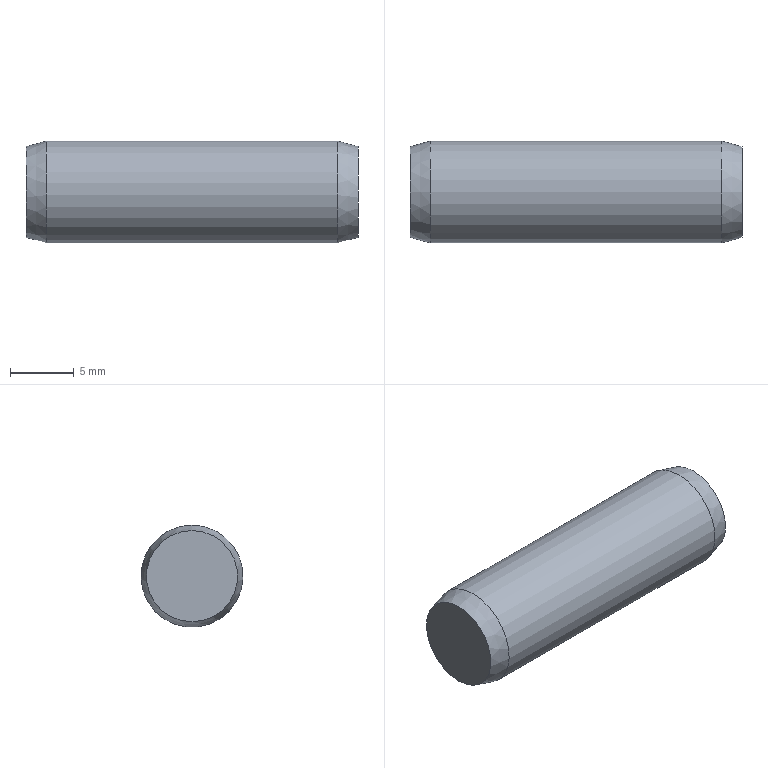Component | NX | GB-T119_1-2000_8X26 | 1 solid | 5 faces | box 26 x 8 x 8 mm | volume 1290 mm3 | plane 2 | cone 2 | cylinder 1 | commonest cylinder face diameters 8 x1
STEP:
#1=CARTESIAN_POINT('',(0.,0.,0.));
#2=DIRECTION('',(0.,0.,1.));
#3=DIRECTION('',(1.,0.,0.));
#4=AXIS2_PLACEMENT_3D('',#1,#2,#3);
#5=CARTESIAN_POINT('',(-11.39,31.008,-213.802));
#6=VERTEX_POINT('',#5);
#7=CARTESIAN_POINT('',(-11.39,31.008,-217.373));
#8=DIRECTION('',(-1.,0.,0.));
#9=DIRECTION('',(0.,0.,1.));
#10=AXIS2_PLACEMENT_3D('',#7,#8,#9);
#11=CIRCLE('',#10,3.571);
#12=CARTESIAN_POINT('',(-11.39,31.008,-217.373));
#13=DIRECTION('',(-1.,0.,0.));
#14=DIRECTION('',(0.,0.,1.));
#15=AXIS2_PLACEMENT_3D('',#12,#13,#14);
#16=PLANE('',#15);
#17=CARTESIAN_POINT('',(0.,0.));
#18=DIRECTION('',(1.,0.));
#19=AXIS2_PLACEMENT_2D('',#17,#18);
#20=CIRCLE('',#19,3.571);
#21=(GEOMETRIC_REPRESENTATION_CONTEXT(2)PARAMETRIC_REPRESENTATION_CONTEXT()REPRESENTATION_CONTEXT('',''));
#22=DEFINITIONAL_REPRESENTATION('',(#20),#21);
#23=PCURVE('',#16,#22);
#24=CARTESIAN_POINT('',(-11.39,31.008,-217.373));
#25=DIRECTION('',(1.,0.,0.));
#26=DIRECTION('',(0.,0.,-1.));
#27=AXIS2_PLACEMENT_3D('',#24,#25,#26);
#28=CONICAL_SURFACE('',#27,3.571,0.2618);
#29=CARTESIAN_POINT('',(9.425,-0.));
#30=DIRECTION('',(-1.,0.));
#31=VECTOR('',#30,1.);
#32=LINE('',#29,#31);
#33=(GEOMETRIC_REPRESENTATION_CONTEXT(2)PARAMETRIC_REPRESENTATION_CONTEXT()REPRESENTATION_CONTEXT('',''));
#34=DEFINITIONAL_REPRESENTATION('',(#32),#33);
#35=PCURVE('',#28,#34);
#36=SURFACE_CURVE('',#11,(#23,#35),.PCURVE_S1.);
#37=EDGE_CURVE('',#6,#6,#36,.T.);
#38=ORIENTED_EDGE('',*,*,#37,.T.);
#39=EDGE_LOOP('',(#38));
#40=FACE_BOUND('',#39,.T.);
#41=ADVANCED_FACE('',(#40),#16,.T.);
#42=CARTESIAN_POINT('',(-9.79,31.008,-213.373));
#43=VERTEX_POINT('',#42);
#44=CARTESIAN_POINT('',(-9.79,31.008,-217.373));
#45=DIRECTION('',(-1.,0.,0.));
#46=DIRECTION('',(0.,0.,1.));
#47=AXIS2_PLACEMENT_3D('',#44,#45,#46);
#48=CIRCLE('',#47,4.);
#49=CARTESIAN_POINT('',(9.425,1.6));
#50=DIRECTION('',(-1.,0.));
#51=VECTOR('',#50,1.);
#52=LINE('',#49,#51);
#53=(GEOMETRIC_REPRESENTATION_CONTEXT(2)PARAMETRIC_REPRESENTATION_CONTEXT()REPRESENTATION_CONTEXT('',''));
#54=DEFINITIONAL_REPRESENTATION('',(#52),#53);
#55=PCURVE('',#28,#54);
#56=CARTESIAN_POINT('',(14.61,31.008,-217.373));
#57=DIRECTION('',(-1.,0.,0.));
#58=DIRECTION('',(0.,0.,1.));
#59=AXIS2_PLACEMENT_3D('',#56,#57,#58);
#60=CYLINDRICAL_SURFACE('',#59,4.);
#61=CARTESIAN_POINT('',(0.,24.4));
#62=DIRECTION('',(1.,0.));
#63=VECTOR('',#62,1.);
#64=LINE('',#61,#63);
#65=(GEOMETRIC_REPRESENTATION_CONTEXT(2)PARAMETRIC_REPRESENTATION_CONTEXT()REPRESENTATION_CONTEXT('',''));
#66=DEFINITIONAL_REPRESENTATION('',(#64),#65);
#67=PCURVE('',#60,#66);
#68=SURFACE_CURVE('',#48,(#55,#67),.PCURVE_S1.);
#69=EDGE_CURVE('',#43,#43,#68,.T.);
#70=ORIENTED_EDGE('',*,*,#69,.T.);
#71=CARTESIAN_POINT('',(-11.39,31.008,-213.802));
#72=CARTESIAN_POINT('',(-9.79,31.008,-213.373));
#73=B_SPLINE_CURVE_WITH_KNOTS('',1,(#71,#72),.UNSPECIFIED.,.F.,.F.,(2,2),(-0.,1.656),.PIECEWISE_BEZIER_KNOTS.);
#74=CARTESIAN_POINT('',(3.142,0.));
#75=DIRECTION('',(0.,1.));
#76=VECTOR('',#75,1.);
#77=LINE('',#74,#76);
#78=(GEOMETRIC_REPRESENTATION_CONTEXT(2)PARAMETRIC_REPRESENTATION_CONTEXT()REPRESENTATION_CONTEXT('',''));
#79=DEFINITIONAL_REPRESENTATION('',(#77),#78);
#80=PCURVE('',#28,#79);
#81=CARTESIAN_POINT('',(9.425,0.));
#82=DIRECTION('',(0.,1.));
#83=VECTOR('',#82,1.);
#84=LINE('',#81,#83);
#85=(GEOMETRIC_REPRESENTATION_CONTEXT(2)PARAMETRIC_REPRESENTATION_CONTEXT()REPRESENTATION_CONTEXT('',''));
#86=DEFINITIONAL_REPRESENTATION('',(#84),#85);
#87=PCURVE('',#28,#86);
#88=SEAM_CURVE('',#73,(#80,#87),.PCURVE_S1.);
#89=EDGE_CURVE('',#6,#43,#88,.T.);
#90=ORIENTED_EDGE('',*,*,#89,.F.);
#91=ORIENTED_EDGE('',*,*,#37,.F.);
#92=ORIENTED_EDGE('',*,*,#89,.T.);
#93=EDGE_LOOP('',(#70,#90,#91,#92));
#94=FACE_BOUND('',#93,.T.);
#95=ADVANCED_FACE('',(#94),#28,.T.);
#96=CARTESIAN_POINT('',(13.01,31.008,-213.373));
#97=VERTEX_POINT('',#96);
#98=CARTESIAN_POINT('',(13.01,31.008,-217.373));
#99=DIRECTION('',(-1.,0.,0.));
#100=DIRECTION('',(0.,0.,1.));
#101=AXIS2_PLACEMENT_3D('',#98,#99,#100);
#102=CIRCLE('',#101,4.);
#103=CARTESIAN_POINT('',(0.,1.6));
#104=DIRECTION('',(1.,0.));
#105=VECTOR('',#104,1.);
#106=LINE('',#103,#105);
#107=(GEOMETRIC_REPRESENTATION_CONTEXT(2)PARAMETRIC_REPRESENTATION_CONTEXT()REPRESENTATION_CONTEXT('',''));
#108=DEFINITIONAL_REPRESENTATION('',(#106),#107);
#109=PCURVE('',#60,#108);
#110=CARTESIAN_POINT('',(13.01,31.008,-217.373));
#111=DIRECTION('',(-1.,0.,0.));
#112=DIRECTION('',(0.,0.,1.));
#113=AXIS2_PLACEMENT_3D('',#110,#111,#112);
#114=CONICAL_SURFACE('',#113,4.,0.2618);
#115=CARTESIAN_POINT('',(0.,-0.));
#116=DIRECTION('',(1.,0.));
#117=VECTOR('',#116,1.);
#118=LINE('',#115,#117);
#119=(GEOMETRIC_REPRESENTATION_CONTEXT(2)PARAMETRIC_REPRESENTATION_CONTEXT()REPRESENTATION_CONTEXT('',''));
#120=DEFINITIONAL_REPRESENTATION('',(#118),#119);
#121=PCURVE('',#114,#120);
#122=SURFACE_CURVE('',#102,(#109,#121),.PCURVE_S1.);
#123=EDGE_CURVE('',#97,#97,#122,.T.);
#124=ORIENTED_EDGE('',*,*,#123,.T.);
#125=CARTESIAN_POINT('',(13.01,31.008,-213.373));
#126=CARTESIAN_POINT('',(-9.79,31.008,-213.373));
#127=B_SPLINE_CURVE_WITH_KNOTS('',1,(#125,#126),.UNSPECIFIED.,.F.,.F.,(2,2),(1.6,24.4),.PIECEWISE_BEZIER_KNOTS.);
#128=CARTESIAN_POINT('',(6.283,0.));
#129=DIRECTION('',(0.,1.));
#130=VECTOR('',#129,1.);
#131=LINE('',#128,#130);
#132=(GEOMETRIC_REPRESENTATION_CONTEXT(2)PARAMETRIC_REPRESENTATION_CONTEXT()REPRESENTATION_CONTEXT('',''));
#133=DEFINITIONAL_REPRESENTATION('',(#131),#132);
#134=PCURVE('',#60,#133);
#135=CARTESIAN_POINT('',(0.,0.));
#136=DIRECTION('',(0.,1.));
#137=VECTOR('',#136,1.);
#138=LINE('',#135,#137);
#139=(GEOMETRIC_REPRESENTATION_CONTEXT(2)PARAMETRIC_REPRESENTATION_CONTEXT()REPRESENTATION_CONTEXT('',''));
#140=DEFINITIONAL_REPRESENTATION('',(#138),#139);
#141=PCURVE('',#60,#140);
#142=SEAM_CURVE('',#127,(#134,#141),.PCURVE_S1.);
#143=EDGE_CURVE('',#97,#43,#142,.T.);
#144=ORIENTED_EDGE('',*,*,#143,.T.);
#145=ORIENTED_EDGE('',*,*,#69,.F.);
#146=ORIENTED_EDGE('',*,*,#143,.F.);
#147=EDGE_LOOP('',(#124,#144,#145,#146));
#148=FACE_BOUND('',#147,.T.);
#149=ADVANCED_FACE('',(#148),#60,.T.);
#150=CARTESIAN_POINT('',(14.61,31.008,-213.802));
#151=VERTEX_POINT('',#150);
#152=CARTESIAN_POINT('',(14.61,31.008,-217.373));
#153=DIRECTION('',(-1.,0.,0.));
#154=DIRECTION('',(0.,0.,1.));
#155=AXIS2_PLACEMENT_3D('',#152,#153,#154);
#156=CIRCLE('',#155,3.571);
#157=CARTESIAN_POINT('',(0.,-1.6));
#158=DIRECTION('',(1.,0.));
#159=VECTOR('',#158,1.);
#160=LINE('',#157,#159);
#161=(GEOMETRIC_REPRESENTATION_CONTEXT(2)PARAMETRIC_REPRESENTATION_CONTEXT()REPRESENTATION_CONTEXT('',''));
#162=DEFINITIONAL_REPRESENTATION('',(#160),#161);
#163=PCURVE('',#114,#162);
#164=CARTESIAN_POINT('',(14.61,31.008,-220.944));
#165=DIRECTION('',(1.,0.,0.));
#166=DIRECTION('',(0.,0.,-1.));
#167=AXIS2_PLACEMENT_3D('',#164,#165,#166);
#168=PLANE('',#167);
#169=CARTESIAN_POINT('',(-7.143,0.));
#170=CARTESIAN_POINT('',(-7.143,6.186));
#171=CARTESIAN_POINT('',(-1.786,3.093));
#172=CARTESIAN_POINT('',(3.571,0.));
#173=CARTESIAN_POINT('',(-1.786,-3.093));
#174=CARTESIAN_POINT('',(-7.143,-6.186));
#175=CARTESIAN_POINT('',(-7.143,0.));
#176=(BOUNDED_CURVE()B_SPLINE_CURVE(2,(#169,#170,#171,#172,#173,#174,#175),.UNSPECIFIED.,.T.,.F.)B_SPLINE_CURVE_WITH_KNOTS((1,2,2,2,2,1),(-2.094,0.,2.094,4.189,6.283,8.378),.UNSPECIFIED.)CURVE()GEOMETRIC_REPRESENTATION_ITEM()RATIONAL_B_SPLINE_CURVE((1.,0.5,1.,0.5,1.,0.5,1.))REPRESENTATION_ITEM(''));
#177=(GEOMETRIC_REPRESENTATION_CONTEXT(2)PARAMETRIC_REPRESENTATION_CONTEXT()REPRESENTATION_CONTEXT('',''));
#178=DEFINITIONAL_REPRESENTATION('',(#176),#177);
#179=PCURVE('',#168,#178);
#180=SURFACE_CURVE('',#156,(#163,#179),.PCURVE_S1.);
#181=EDGE_CURVE('',#151,#151,#180,.T.);
#182=ORIENTED_EDGE('',*,*,#181,.T.);
#183=CARTESIAN_POINT('',(14.61,31.008,-213.802));
#184=CARTESIAN_POINT('',(13.01,31.008,-213.373));
#185=B_SPLINE_CURVE_WITH_KNOTS('',1,(#183,#184),.UNSPECIFIED.,.F.,.F.,(2,2),(-1.656,-0.),.PIECEWISE_BEZIER_KNOTS.);
#186=CARTESIAN_POINT('',(6.283,0.));
#187=DIRECTION('',(0.,1.));
#188=VECTOR('',#187,1.);
#189=LINE('',#186,#188);
#190=(GEOMETRIC_REPRESENTATION_CONTEXT(2)PARAMETRIC_REPRESENTATION_CONTEXT()REPRESENTATION_CONTEXT('',''));
#191=DEFINITIONAL_REPRESENTATION('',(#189),#190);
#192=PCURVE('',#114,#191);
#193=CARTESIAN_POINT('',(0.,0.));
#194=DIRECTION('',(0.,1.));
#195=VECTOR('',#194,1.);
#196=LINE('',#193,#195);
#197=(GEOMETRIC_REPRESENTATION_CONTEXT(2)PARAMETRIC_REPRESENTATION_CONTEXT()REPRESENTATION_CONTEXT('',''));
#198=DEFINITIONAL_REPRESENTATION('',(#196),#197);
#199=PCURVE('',#114,#198);
#200=SEAM_CURVE('',#185,(#192,#199),.PCURVE_S1.);
#201=EDGE_CURVE('',#151,#97,#200,.T.);
#202=ORIENTED_EDGE('',*,*,#201,.T.);
#203=ORIENTED_EDGE('',*,*,#123,.F.);
#204=ORIENTED_EDGE('',*,*,#201,.F.);
#205=EDGE_LOOP('',(#182,#202,#203,#204));
#206=FACE_BOUND('',#205,.T.);
#207=ADVANCED_FACE('',(#206),#114,.T.);
#208=ORIENTED_EDGE('',*,*,#181,.F.);
#209=EDGE_LOOP('',(#208));
#210=FACE_BOUND('',#209,.T.);
#211=ADVANCED_FACE('',(#210),#168,.T.);
#212=CLOSED_SHELL('',(#41,#95,#149,#207,#211));
#213=MANIFOLD_SOLID_BREP('',#212);
#214=(LENGTH_UNIT()NAMED_UNIT(*)SI_UNIT(.MILLI.,.METRE.));
#215=UNCERTAINTY_MEASURE_WITH_UNIT(LENGTH_MEASURE(0.00001),#214,'','');
#216=(NAMED_UNIT(*)PLANE_ANGLE_UNIT()SI_UNIT($,.RADIAN.));
#217=(NAMED_UNIT(*)SI_UNIT($,.STERADIAN.)SOLID_ANGLE_UNIT());
#218=(GEOMETRIC_REPRESENTATION_CONTEXT(3)GLOBAL_UNCERTAINTY_ASSIGNED_CONTEXT((#215))GLOBAL_UNIT_ASSIGNED_CONTEXT((#214,#216,#217))REPRESENTATION_CONTEXT('',''));
#219=ADVANCED_BREP_SHAPE_REPRESENTATION('',(#4,#213),#218);